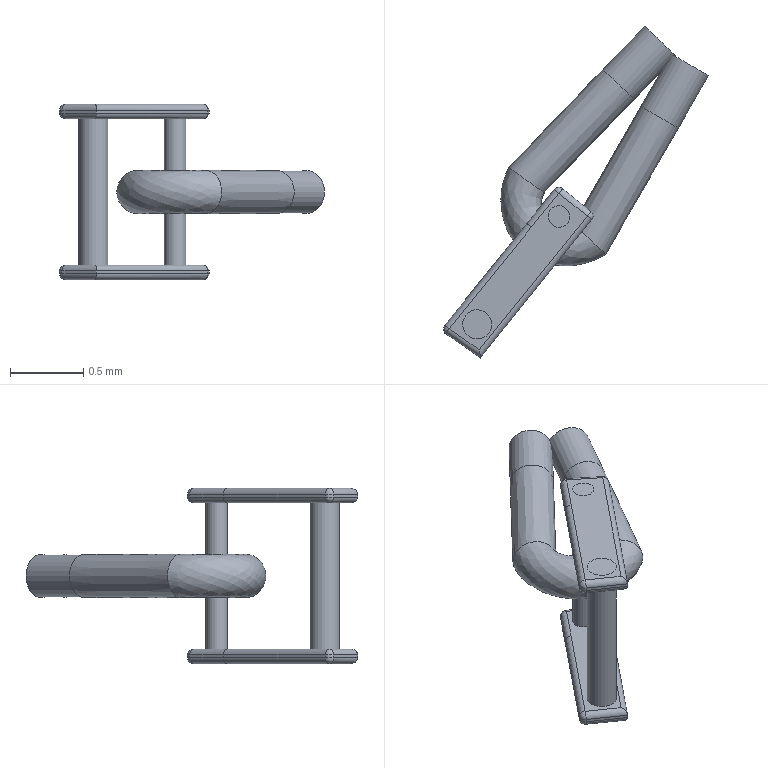Component | NX | MODEL11_3 | 5 solids | 70 faces | volume 0 mm3 | cylinder 35 | plane 20 | sphere 12 | spline 3 | commonest cylinder face diameters 0.08 x26 0.148 x4 0.2 x3 0.296 x2